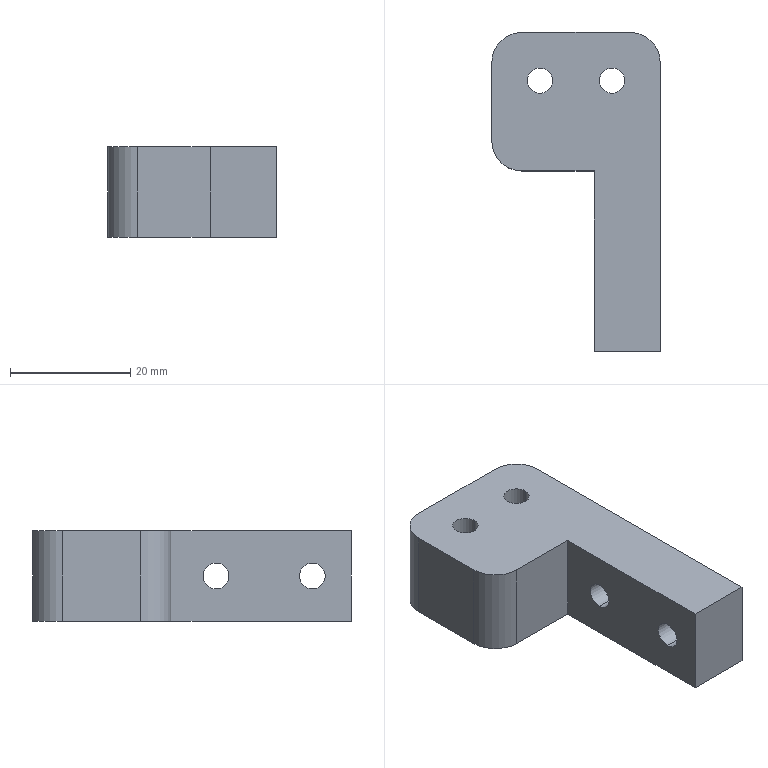CAM job | Mastercam | mm | 13 operations | part box 28 x 53 x 15
1. Facing | 20 - 63 平铣刀
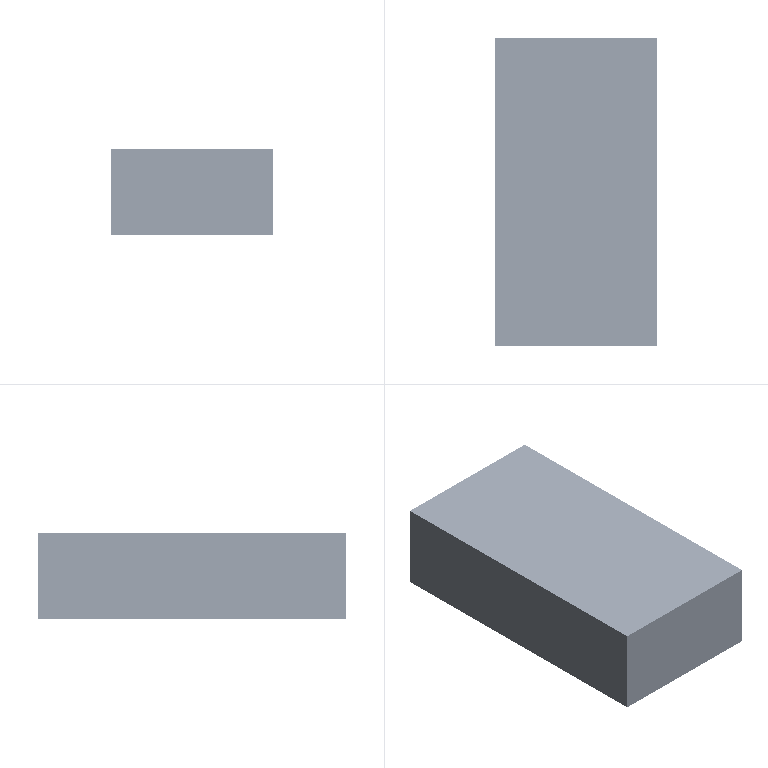2. Contour (Ramp) | 9 - 10 平铣刀
3. Contour (2D) | 10 - 10 平铣刀
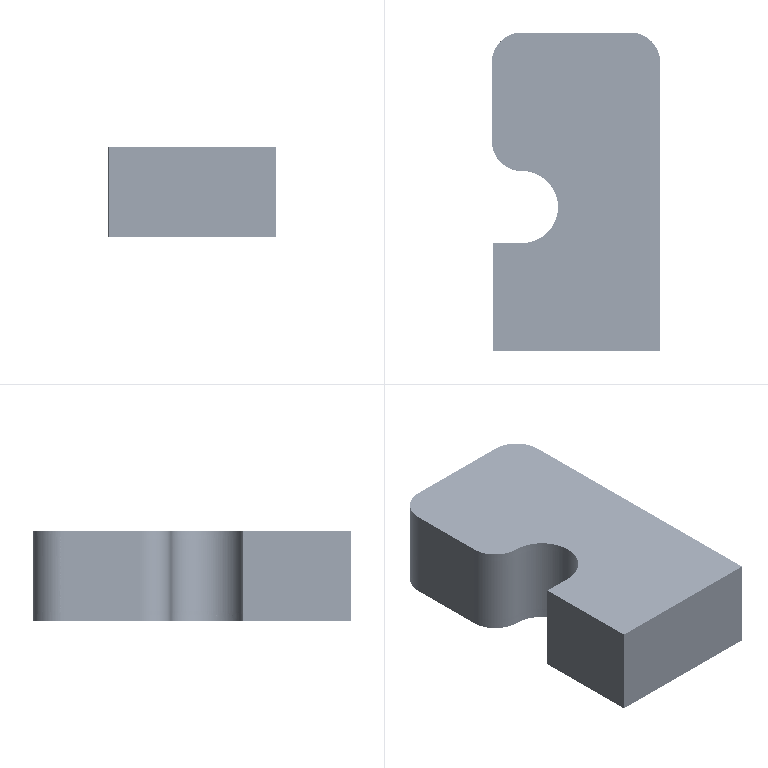4. Contour (2D chamfer) | 7 - 4 倒角刀
5. Drill/Counterbore | 7 - 4 倒角刀
6. Facing | 20 - 63 平铣刀
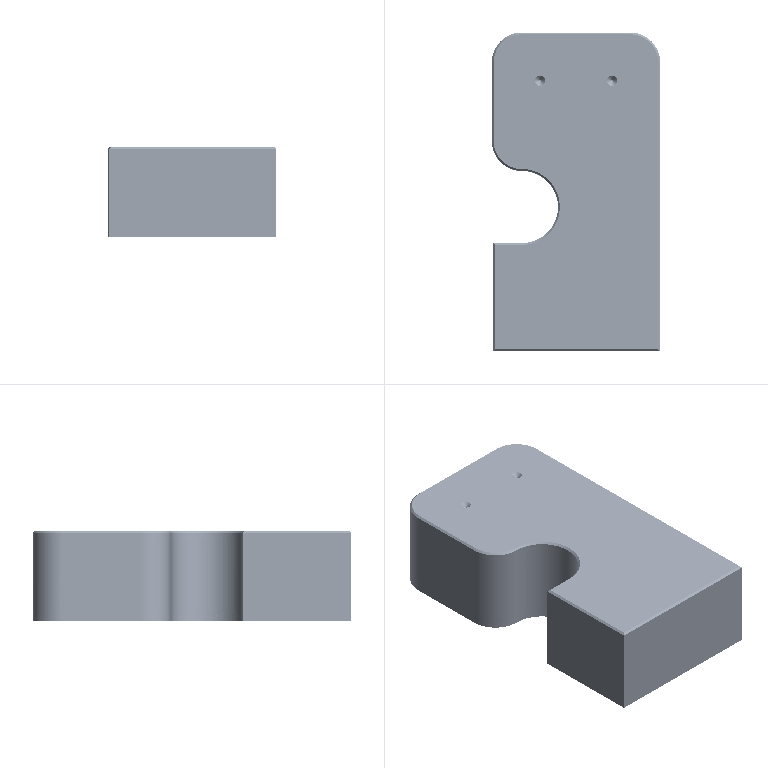7. Contour (2D chamfer) | 7 - 4 倒角刀
8. Helix Bore | 4 - 4 平铣刀
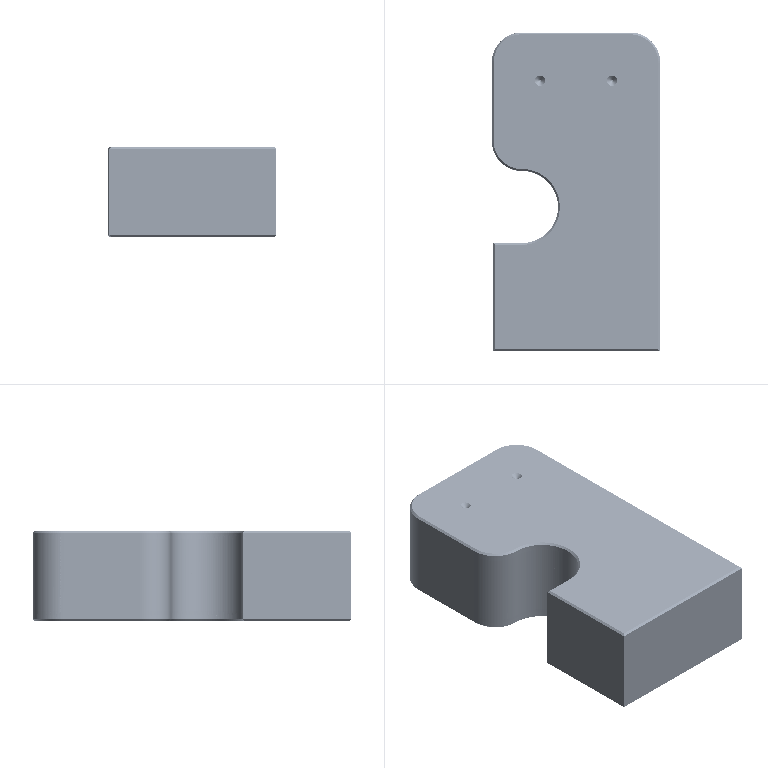9. Contour (2D chamfer) | 7 - 4 倒角刀
10. Contour (2D) | 9 - 10 平铣刀
11. Contour (2D) | 10 - 10 平铣刀
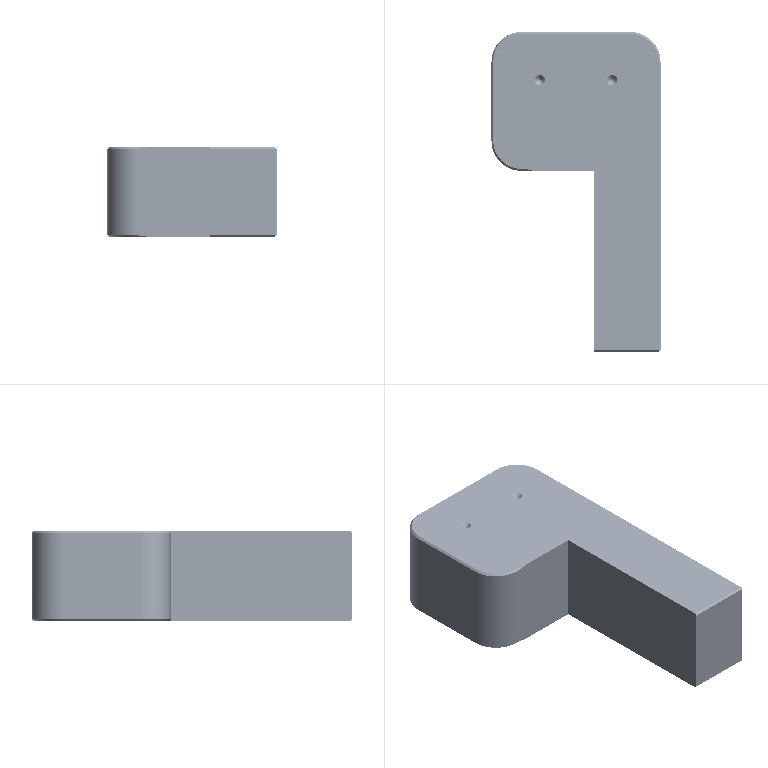12. Drill/Counterbore | 7 - 4 倒角刀
13. Contour (2D chamfer) | 7 - 4 倒角刀